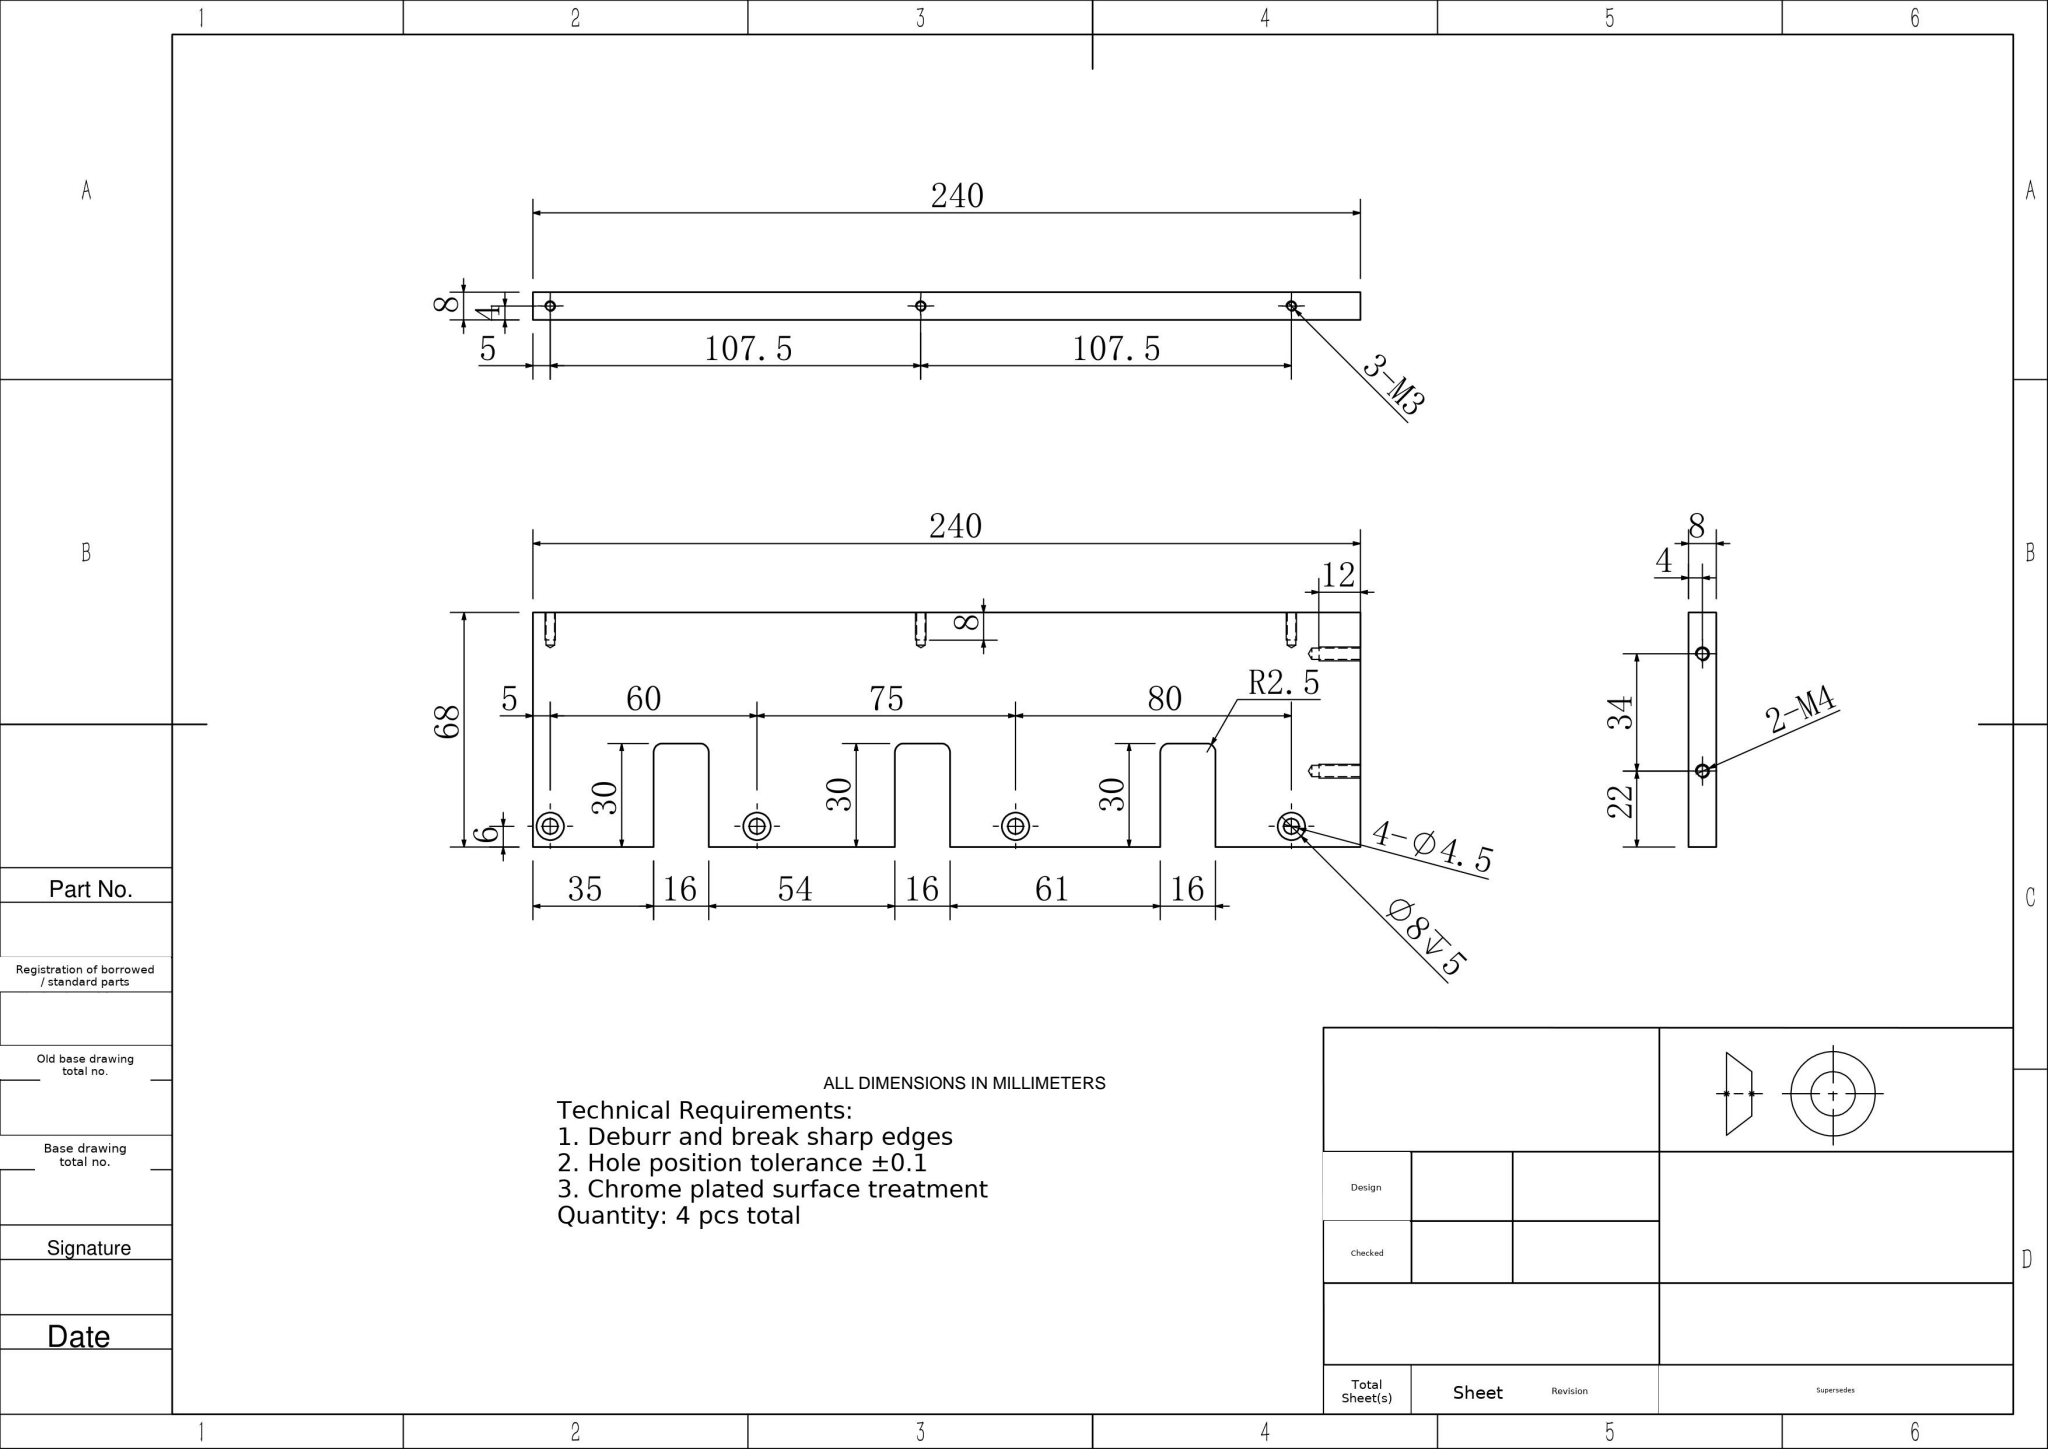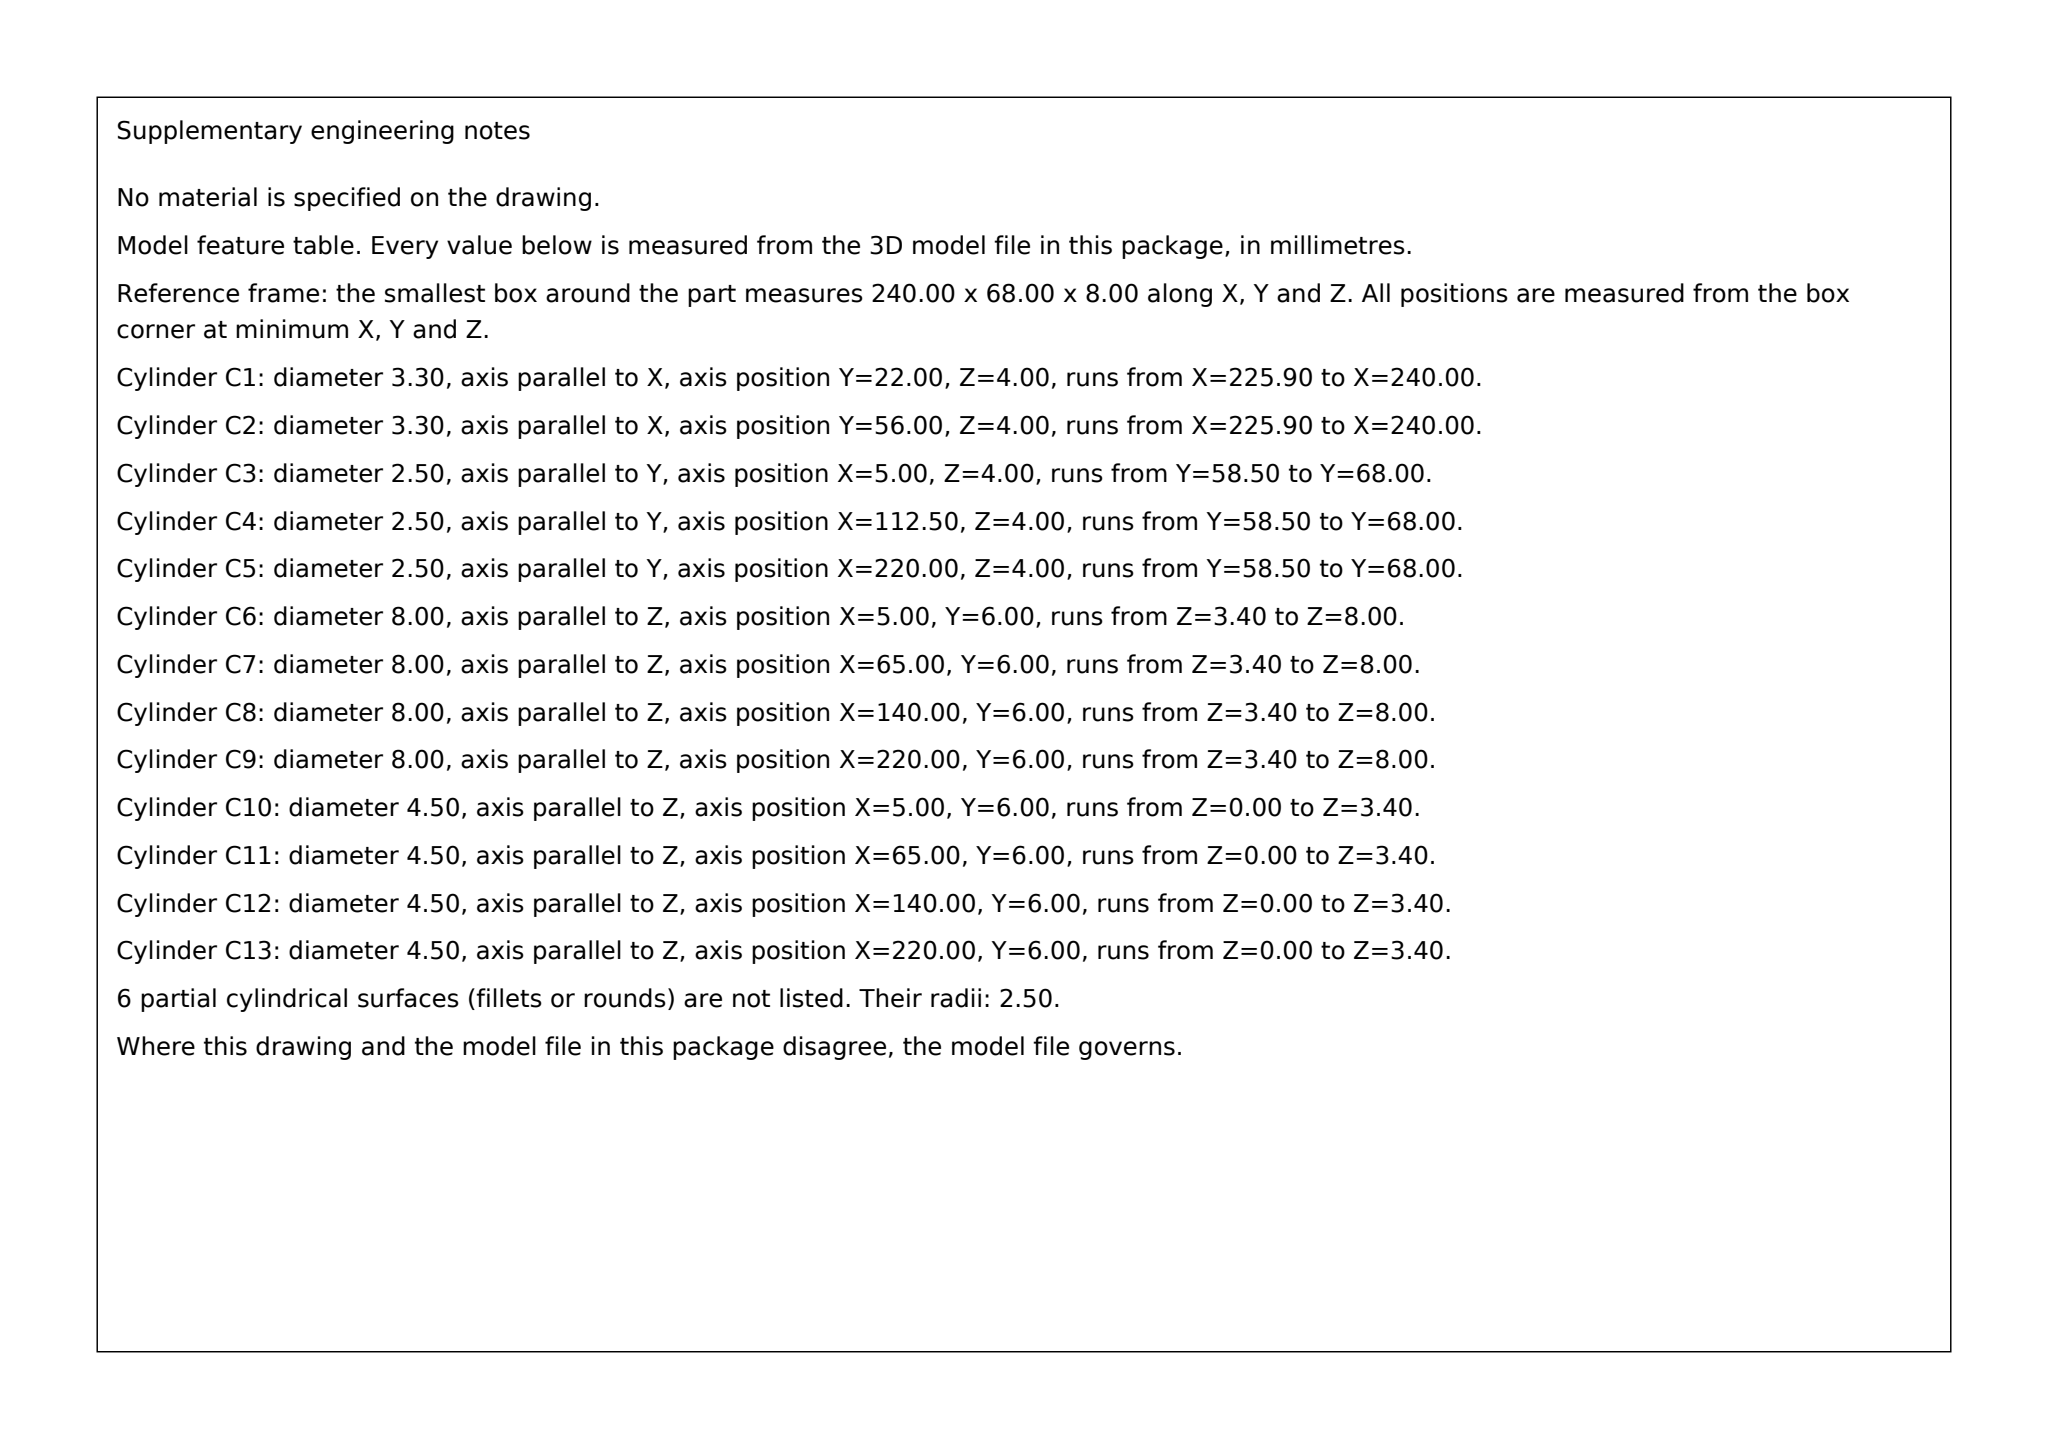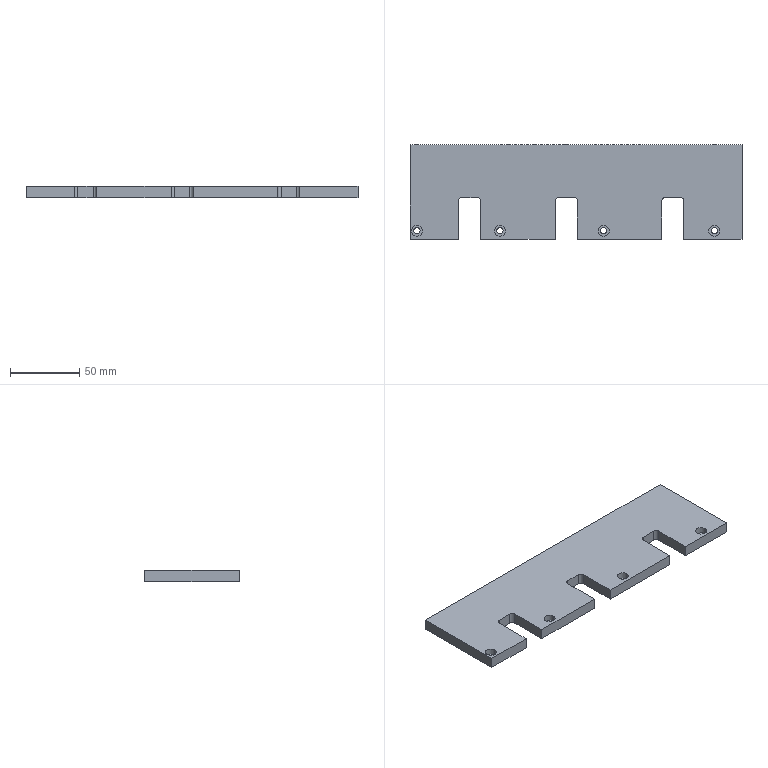Part | SolidWorks | mm | 1 solid | 64 faces | box 240 x 68 x 8 mm | volume 117573 mm3 | cylinder 32 | plane 22 | cone 10 | commonest cylinder face diameters 8 x8 4.5 x8 2.5 x6 5 x6 3.3 x4
build123d program:
from build123d import *

# Parameters (mm, degrees)
SKETCH1_W                                         = 240
SKETCH1_H                                         = 68
BOSS_EXTRUDE1_DEPTH                               = 4
M3_TAPPED_HOLE1_D                                 = 2.5
M3_TAPPED_HOLE1_DEPTH                             = 9.5
M3_TAPPED_HOLE1_TIP                               = 0.7511
HOLE_SIZE_ACCORDING_TO_HEXAGON_SOCKET_D           = 4.5
HOLE_SIZE_ACCORDING_TO_HEXAGON_SOCKET_CBORE_D     = 8
HOLE_SIZE_ACCORDING_TO_HEXAGON_SOCKET_CBORE_DEPTH = 4.6
SKETCH6_W                                         = 16
SKETCH6_H                                         = 30
CUT_EXTRUDE1_DEPTH                                = 125.98
M4_TAPPED_HOLE1_D                                 = 3.3
M4_TAPPED_HOLE1_DEPTH                             = 14.1
M4_TAPPED_HOLE1_TIP                               = 0.9914
FILLET1_R                                         = 2.5


with BuildPart() as part:
    # Sketch1 → Boss-Extrude1 (new, symmetric)
    with BuildSketch(Plane.XY):
        Rectangle(SKETCH1_W, SKETCH1_H)
    extrude(amount=BOSS_EXTRUDE1_DEPTH, both=True)

    # M3 Tapped Hole1
    with Locations(Plane(origin=(0, 34, 0), x_dir=(1, 0, 0), z_dir=(0, 1, 0))):
        with Locations((-115, 0), (-7.5, 0), (100, 0)):
            Hole(M3_TAPPED_HOLE1_D / 2, depth=M3_TAPPED_HOLE1_DEPTH)
            with Locations((0, 0, -(M3_TAPPED_HOLE1_DEPTH + M3_TAPPED_HOLE1_TIP / 2))):  # 118° drill point
                Cone(0, M3_TAPPED_HOLE1_D / 2, M3_TAPPED_HOLE1_TIP, mode=Mode.SUBTRACT)

    # Hole Size _ according to_ Hexagon Socket (through all)
    with Locations(Plane.XY.offset(4)):
        with Locations((-115, -28), (-55, -28), (20, -28), (100, -28)):
            CounterBoreHole(HOLE_SIZE_ACCORDING_TO_HEXAGON_SOCKET_D / 2, HOLE_SIZE_ACCORDING_TO_HEXAGON_SOCKET_CBORE_D / 2, HOLE_SIZE_ACCORDING_TO_HEXAGON_SOCKET_CBORE_DEPTH)

    # Sketch6 → Cut-Extrude1 (cut, through all)
    with BuildSketch(Plane.XY.offset(4)):
        with Locations((-77, -19)):
            Rectangle(SKETCH6_W, SKETCH6_H)
        with Locations((-7, -19)):
            Rectangle(SKETCH6_W, SKETCH6_H)
        with Locations((70, -19)):
            Rectangle(SKETCH6_W, SKETCH6_H)
    extrude(amount=-CUT_EXTRUDE1_DEPTH, mode=Mode.SUBTRACT)

    # M4 Tapped Hole1
    with Locations(Plane(origin=(120, 0, 0), x_dir=(0, 0, -1), z_dir=(1, 0, 0))):
        with Locations((0, 22), (0, -12)):
            Hole(M4_TAPPED_HOLE1_D / 2, depth=M4_TAPPED_HOLE1_DEPTH)
            with Locations((0, 0, -(M4_TAPPED_HOLE1_DEPTH + M4_TAPPED_HOLE1_TIP / 2))):  # 118° drill point
                Cone(0, M4_TAPPED_HOLE1_D / 2, M4_TAPPED_HOLE1_TIP, mode=Mode.SUBTRACT)

    # Fillet1
    fillet1_edges = [part.edges().sort_by_distance(p)[0] for p in [
        (-85, -4, 0),
        (-69, -4, 0),
        (-15, -4, 0),
        (1, -4, 0),
        (62, -4, 0),
        (78, -4, 0),
    ]]
    fillet(fillet1_edges, radius=FILLET1_R)


solid = part.part